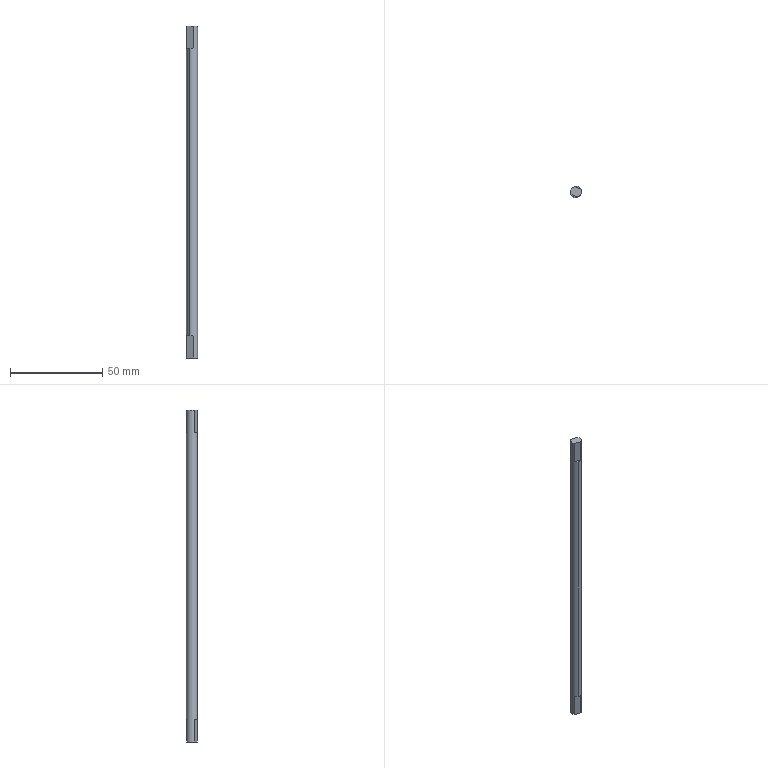Component | SolidWorks | PryBarAxis.1-1 | 1 solid | 12 faces | box 6 x 6 x 180 mm | volume 4991 mm3 | plane 10 | cylinder 2 | commonest cylinder face diameters 6 x2
build123d program:
from build123d import *

# Parameters (mm, degrees)
SKETCH1_R           = 3
BOSS_EXTRUDE1_DEPTH = 180
SKETCH2_W           = 1.83
SKETCH2_H           = 6.945
SKETCH2_W_2         = 2.107
CUT_EXTRUDE1_DEPTH  = 12
SKETCH3_W           = 1.492
SKETCH3_H           = 3.969
SKETCH3_W_2         = 1.313
CUT_EXTRUDE2_DEPTH  = 12


with BuildPart() as part:
    # Sketch1 → Boss-Extrude1 (new body)
    with BuildSketch(Plane.XY):
        with Locations(Location((0, 0, 0), (0, 0, 180))):
            Circle(SKETCH1_R)
    extrude(amount=BOSS_EXTRUDE1_DEPTH)

    # Sketch2 → Cut-Extrude1 (cut)
    with BuildSketch(Plane.XY.offset(180)):
        with Locations((-3.165, 0.1105)):
            Rectangle(SKETCH2_W, SKETCH2_H)
        with Locations((3.303, 0.1105)):
            Rectangle(SKETCH2_W_2, SKETCH2_H)
    extrude(amount=-CUT_EXTRUDE1_DEPTH, mode=Mode.SUBTRACT)

    # Sketch3 → Cut-Extrude2 (cut)
    with BuildSketch(Plane(origin=(0, 0, 0), x_dir=(-1, 0, 0), z_dir=(0, 0, -1))):
        with Locations((2.996, 0)):
            Rectangle(SKETCH3_W, SKETCH3_H)
        with Locations((-2.906, 0)):
            Rectangle(SKETCH3_W_2, SKETCH3_H)
    extrude(amount=-CUT_EXTRUDE2_DEPTH, mode=Mode.SUBTRACT)


solid = part.part

# Placed as in the assembly
solid = solid.moved(Location((65, 200, 90), (-180, 0, -66.765)))
STEP:
#1=COLOUR_RGB('',0.7922,0.8196,0.9333);
#2=FILL_AREA_STYLE_COLOUR('',#1);
#3=FILL_AREA_STYLE('',(#2));
#4=SURFACE_STYLE_FILL_AREA(#3);
#5=SURFACE_SIDE_STYLE('',(#4));
#6=SURFACE_STYLE_USAGE(.BOTH.,#5);
#7=PRESENTATION_STYLE_ASSIGNMENT((#6));
#8=CARTESIAN_POINT('',(2.512,7.765,3.071));
#9=VERTEX_POINT('',#8);
#10=CARTESIAN_POINT('',(2.596,7.762,3.071));
#11=VERTEX_POINT('',#10);
#12=CARTESIAN_POINT('',(2.559,7.874,3.071));
#13=DIRECTION('',(0.,0.,1.));
#14=DIRECTION('',(-0.3945,-0.9189,0.));
#15=AXIS2_PLACEMENT_3D('',#12,#13,#14);
#16=CIRCLE('',#15,0.1181);
#17=EDGE_CURVE('',#9,#11,#16,.T.);
#18=ORIENTED_EDGE('',*,*,#17,.F.);
#19=CARTESIAN_POINT('',(2.512,7.765,-3.071));
#20=VERTEX_POINT('',#19);
#21=CARTESIAN_POINT('',(2.512,7.765,3.543));
#22=DIRECTION('',(0.,0.,-1.));
#23=VECTOR('',#22,39.37);
#24=LINE('',#21,#23);
#25=EDGE_CURVE('',#9,#20,#24,.T.);
#26=ORIENTED_EDGE('',*,*,#25,.T.);
#27=CARTESIAN_POINT('',(2.596,7.762,-3.071));
#28=VERTEX_POINT('',#27);
#29=CARTESIAN_POINT('',(2.559,7.874,-3.071));
#30=DIRECTION('',(0.,0.,-1.));
#31=DIRECTION('',(0.3945,0.9189,0.));
#32=AXIS2_PLACEMENT_3D('',#29,#30,#31);
#33=CIRCLE('',#32,0.1181);
#34=EDGE_CURVE('',#28,#20,#33,.T.);
#35=ORIENTED_EDGE('',*,*,#34,.F.);
#36=CARTESIAN_POINT('',(2.596,7.762,-3.543));
#37=VERTEX_POINT('',#36);
#38=CARTESIAN_POINT('',(2.596,7.762,-3.071));
#39=DIRECTION('',(0.,0.,-1.));
#40=VECTOR('',#39,39.37);
#41=LINE('',#38,#40);
#42=EDGE_CURVE('',#28,#37,#41,.T.);
#43=ORIENTED_EDGE('',*,*,#42,.T.);
#44=CARTESIAN_POINT('',(2.666,7.925,-3.543));
#45=VERTEX_POINT('',#44);
#46=CARTESIAN_POINT('',(2.559,7.874,-3.543));
#47=DIRECTION('',(0.,0.,1.));
#48=DIRECTION('',(-0.3945,-0.9189,0.));
#49=AXIS2_PLACEMENT_3D('',#46,#47,#48);
#50=CIRCLE('',#49,0.1181);
#51=EDGE_CURVE('',#37,#45,#50,.T.);
#52=ORIENTED_EDGE('',*,*,#51,.T.);
#53=CARTESIAN_POINT('',(2.666,7.925,-3.071));
#54=VERTEX_POINT('',#53);
#55=CARTESIAN_POINT('',(2.666,7.925,-3.071));
#56=DIRECTION('',(0.,0.,-1.));
#57=VECTOR('',#56,39.37);
#58=LINE('',#55,#57);
#59=EDGE_CURVE('',#54,#45,#58,.T.);
#60=ORIENTED_EDGE('',*,*,#59,.F.);
#61=CARTESIAN_POINT('',(2.606,7.983,-3.071));
#62=VERTEX_POINT('',#61);
#63=CARTESIAN_POINT('',(2.559,7.874,-3.071));
#64=DIRECTION('',(0.,0.,1.));
#65=DIRECTION('',(-0.3945,-0.9189,0.));
#66=AXIS2_PLACEMENT_3D('',#63,#64,#65);
#67=CIRCLE('',#66,0.1181);
#68=EDGE_CURVE('',#54,#62,#67,.T.);
#69=ORIENTED_EDGE('',*,*,#68,.T.);
#70=CARTESIAN_POINT('',(2.606,7.983,3.071));
#71=VERTEX_POINT('',#70);
#72=CARTESIAN_POINT('',(2.606,7.983,3.543));
#73=DIRECTION('',(0.,0.,-1.));
#74=VECTOR('',#73,39.37);
#75=LINE('',#72,#74);
#76=EDGE_CURVE('',#71,#62,#75,.T.);
#77=ORIENTED_EDGE('',*,*,#76,.F.);
#78=CARTESIAN_POINT('',(2.666,7.925,3.071));
#79=VERTEX_POINT('',#78);
#80=CARTESIAN_POINT('',(2.559,7.874,3.071));
#81=DIRECTION('',(0.,0.,1.));
#82=DIRECTION('',(-0.3945,-0.9189,0.));
#83=AXIS2_PLACEMENT_3D('',#80,#81,#82);
#84=CIRCLE('',#83,0.1181);
#85=EDGE_CURVE('',#79,#71,#84,.T.);
#86=ORIENTED_EDGE('',*,*,#85,.F.);
#87=CARTESIAN_POINT('',(2.666,7.925,3.543));
#88=VERTEX_POINT('',#87);
#89=CARTESIAN_POINT('',(2.666,7.925,3.543));
#90=DIRECTION('',(0.,0.,1.));
#91=VECTOR('',#90,39.37);
#92=LINE('',#89,#91);
#93=EDGE_CURVE('',#79,#88,#92,.T.);
#94=ORIENTED_EDGE('',*,*,#93,.T.);
#95=CARTESIAN_POINT('',(2.596,7.762,3.543));
#96=VERTEX_POINT('',#95);
#97=CARTESIAN_POINT('',(2.559,7.874,3.543));
#98=DIRECTION('',(0.,0.,1.));
#99=DIRECTION('',(-0.3945,-0.9189,0.));
#100=AXIS2_PLACEMENT_3D('',#97,#98,#99);
#101=CIRCLE('',#100,0.1181);
#102=EDGE_CURVE('',#96,#88,#101,.T.);
#103=ORIENTED_EDGE('',*,*,#102,.F.);
#104=CARTESIAN_POINT('',(2.596,7.762,3.543));
#105=DIRECTION('',(0.,0.,-1.));
#106=VECTOR('',#105,39.37);
#107=LINE('',#104,#106);
#108=EDGE_CURVE('',#96,#11,#107,.T.);
#109=ORIENTED_EDGE('',*,*,#108,.T.);
#110=EDGE_LOOP('',(#18,#26,#35,#43,#52,#60,#69,#77,#86,#94,#103,#109));
#111=FACE_OUTER_BOUND('',#110,.T.);
#112=CARTESIAN_POINT('',(2.559,7.874,3.543));
#113=DIRECTION('',(0.,0.,-1.));
#114=DIRECTION('',(0.3945,0.9189,0.));
#115=AXIS2_PLACEMENT_3D('',#112,#113,#114);
#116=CYLINDRICAL_SURFACE('',#115,0.1181);
#117=ADVANCED_FACE('',(#111),#116,.T.);
#118=ORIENTED_EDGE('',*,*,#25,.F.);
#119=CARTESIAN_POINT('',(2.452,7.823,3.071));
#120=VERTEX_POINT('',#119);
#121=CARTESIAN_POINT('',(2.559,7.874,3.071));
#122=DIRECTION('',(0.,0.,1.));
#123=DIRECTION('',(-0.3945,-0.9189,0.));
#124=AXIS2_PLACEMENT_3D('',#121,#122,#123);
#125=CIRCLE('',#124,0.1181);
#126=EDGE_CURVE('',#120,#9,#125,.T.);
#127=ORIENTED_EDGE('',*,*,#126,.F.);
#128=CARTESIAN_POINT('',(2.452,7.823,3.543));
#129=VERTEX_POINT('',#128);
#130=CARTESIAN_POINT('',(2.452,7.823,3.543));
#131=DIRECTION('',(0.,0.,1.));
#132=VECTOR('',#131,39.37);
#133=LINE('',#130,#132);
#134=EDGE_CURVE('',#120,#129,#133,.T.);
#135=ORIENTED_EDGE('',*,*,#134,.T.);
#136=CARTESIAN_POINT('',(2.522,7.986,3.543));
#137=VERTEX_POINT('',#136);
#138=CARTESIAN_POINT('',(2.559,7.874,3.543));
#139=DIRECTION('',(0.,0.,1.));
#140=DIRECTION('',(-0.3945,-0.9189,0.));
#141=AXIS2_PLACEMENT_3D('',#138,#139,#140);
#142=CIRCLE('',#141,0.1181);
#143=EDGE_CURVE('',#137,#129,#142,.T.);
#144=ORIENTED_EDGE('',*,*,#143,.F.);
#145=CARTESIAN_POINT('',(2.522,7.986,3.071));
#146=VERTEX_POINT('',#145);
#147=CARTESIAN_POINT('',(2.522,7.986,3.543));
#148=DIRECTION('',(0.,0.,-1.));
#149=VECTOR('',#148,39.37);
#150=LINE('',#147,#149);
#151=EDGE_CURVE('',#137,#146,#150,.T.);
#152=ORIENTED_EDGE('',*,*,#151,.T.);
#153=CARTESIAN_POINT('',(2.559,7.874,3.071));
#154=DIRECTION('',(0.,0.,1.));
#155=DIRECTION('',(-0.3945,-0.9189,0.));
#156=AXIS2_PLACEMENT_3D('',#153,#154,#155);
#157=CIRCLE('',#156,0.1181);
#158=EDGE_CURVE('',#71,#146,#157,.T.);
#159=ORIENTED_EDGE('',*,*,#158,.F.);
#160=ORIENTED_EDGE('',*,*,#76,.T.);
#161=CARTESIAN_POINT('',(2.522,7.986,-3.071));
#162=VERTEX_POINT('',#161);
#163=CARTESIAN_POINT('',(2.559,7.874,-3.071));
#164=DIRECTION('',(0.,0.,1.));
#165=DIRECTION('',(-0.3945,-0.9189,0.));
#166=AXIS2_PLACEMENT_3D('',#163,#164,#165);
#167=CIRCLE('',#166,0.1181);
#168=EDGE_CURVE('',#62,#162,#167,.T.);
#169=ORIENTED_EDGE('',*,*,#168,.T.);
#170=CARTESIAN_POINT('',(2.522,7.986,-3.543));
#171=VERTEX_POINT('',#170);
#172=CARTESIAN_POINT('',(2.522,7.986,-3.071));
#173=DIRECTION('',(0.,0.,-1.));
#174=VECTOR('',#173,39.37);
#175=LINE('',#172,#174);
#176=EDGE_CURVE('',#162,#171,#175,.T.);
#177=ORIENTED_EDGE('',*,*,#176,.T.);
#178=CARTESIAN_POINT('',(2.452,7.823,-3.543));
#179=VERTEX_POINT('',#178);
#180=CARTESIAN_POINT('',(2.559,7.874,-3.543));
#181=DIRECTION('',(0.,0.,1.));
#182=DIRECTION('',(-0.3945,-0.9189,0.));
#183=AXIS2_PLACEMENT_3D('',#180,#181,#182);
#184=CIRCLE('',#183,0.1181);
#185=EDGE_CURVE('',#171,#179,#184,.T.);
#186=ORIENTED_EDGE('',*,*,#185,.T.);
#187=CARTESIAN_POINT('',(2.452,7.823,-3.071));
#188=VERTEX_POINT('',#187);
#189=CARTESIAN_POINT('',(2.452,7.823,-3.071));
#190=DIRECTION('',(0.,0.,-1.));
#191=VECTOR('',#190,39.37);
#192=LINE('',#189,#191);
#193=EDGE_CURVE('',#188,#179,#192,.T.);
#194=ORIENTED_EDGE('',*,*,#193,.F.);
#195=CARTESIAN_POINT('',(2.559,7.874,-3.071));
#196=DIRECTION('',(0.,0.,-1.));
#197=DIRECTION('',(0.3945,0.9189,0.));
#198=AXIS2_PLACEMENT_3D('',#195,#196,#197);
#199=CIRCLE('',#198,0.1181);
#200=EDGE_CURVE('',#20,#188,#199,.T.);
#201=ORIENTED_EDGE('',*,*,#200,.F.);
#202=EDGE_LOOP('',(#118,#127,#135,#144,#152,#159,#160,#169,#177,#186,#194,#201));
#203=FACE_OUTER_BOUND('',#202,.T.);
#204=CARTESIAN_POINT('',(2.559,7.874,3.543));
#205=DIRECTION('',(0.,0.,-1.));
#206=DIRECTION('',(0.3945,0.9189,0.));
#207=AXIS2_PLACEMENT_3D('',#204,#205,#206);
#208=CYLINDRICAL_SURFACE('',#207,0.1181);
#209=ADVANCED_FACE('',(#203),#208,.T.);
#210=CARTESIAN_POINT('',(2.524,7.793,3.543));
#211=DIRECTION('',(-0.9189,0.3945,0.));
#212=VECTOR('',#211,39.37);
#213=LINE('',#210,#212);
#214=EDGE_CURVE('',#96,#129,#213,.T.);
#215=ORIENTED_EDGE('',*,*,#214,.F.);
#216=ORIENTED_EDGE('',*,*,#102,.T.);
#217=CARTESIAN_POINT('',(2.594,7.955,3.543));
#218=DIRECTION('',(0.9189,-0.3945,0.));
#219=VECTOR('',#218,39.37);
#220=LINE('',#217,#219);
#221=EDGE_CURVE('',#137,#88,#220,.T.);
#222=ORIENTED_EDGE('',*,*,#221,.F.);
#223=ORIENTED_EDGE('',*,*,#143,.T.);
#224=EDGE_LOOP('',(#215,#216,#222,#223));
#225=FACE_OUTER_BOUND('',#224,.T.);
#226=CARTESIAN_POINT('',(2.559,7.874,3.543));
#227=DIRECTION('',(0.,0.,1.));
#228=DIRECTION('',(-0.3945,-0.9189,0.));
#229=AXIS2_PLACEMENT_3D('',#226,#227,#228);
#230=PLANE('',#229);
#231=ADVANCED_FACE('',(#225),#230,.T.);
#232=ORIENTED_EDGE('',*,*,#51,.F.);
#233=CARTESIAN_POINT('',(2.596,7.762,-3.543));
#234=DIRECTION('',(0.9189,-0.3945,0.));
#235=VECTOR('',#234,39.37);
#236=LINE('',#233,#235);
#237=EDGE_CURVE('',#179,#37,#236,.T.);
#238=ORIENTED_EDGE('',*,*,#237,.F.);
#239=ORIENTED_EDGE('',*,*,#185,.F.);
#240=CARTESIAN_POINT('',(2.522,7.986,-3.543));
#241=DIRECTION('',(-0.9189,0.3945,0.));
#242=VECTOR('',#241,39.37);
#243=LINE('',#240,#242);
#244=EDGE_CURVE('',#45,#171,#243,.T.);
#245=ORIENTED_EDGE('',*,*,#244,.F.);
#246=EDGE_LOOP('',(#232,#238,#239,#245));
#247=FACE_OUTER_BOUND('',#246,.T.);
#248=CARTESIAN_POINT('',(2.559,7.874,-3.543));
#249=DIRECTION('',(0.,0.,1.));
#250=DIRECTION('',(-0.3945,-0.9189,0.));
#251=AXIS2_PLACEMENT_3D('',#248,#249,#250);
#252=PLANE('',#251);
#253=ADVANCED_FACE('',(#247),#252,.F.);
#254=ORIENTED_EDGE('',*,*,#85,.T.);
#255=ORIENTED_EDGE('',*,*,#158,.T.);
#256=CARTESIAN_POINT('',(2.724,7.9,3.071));
#257=DIRECTION('',(0.9189,-0.3945,0.));
#258=VECTOR('',#257,39.37);
#259=LINE('',#256,#258);
#260=EDGE_CURVE('',#146,#79,#259,.T.);
#261=ORIENTED_EDGE('',*,*,#260,.T.);
#262=EDGE_LOOP('',(#254,#255,#261));
#263=FACE_OUTER_BOUND('',#262,.T.);
#264=CARTESIAN_POINT('',(2.752,7.966,3.071));
#265=DIRECTION('',(0.,0.,1.));
#266=DIRECTION('',(-0.3945,-0.9189,0.));
#267=AXIS2_PLACEMENT_3D('',#264,#265,#266);
#268=PLANE('',#267);
#269=ADVANCED_FACE('',(#263),#268,.T.);
#270=ORIENTED_EDGE('',*,*,#221,.T.);
#271=ORIENTED_EDGE('',*,*,#93,.F.);
#272=ORIENTED_EDGE('',*,*,#260,.F.);
#273=ORIENTED_EDGE('',*,*,#151,.F.);
#274=EDGE_LOOP('',(#270,#271,#272,#273));
#275=FACE_OUTER_BOUND('',#274,.T.);
#276=CARTESIAN_POINT('',(2.724,7.9,3.071));
#277=DIRECTION('',(-0.3945,-0.9189,0.));
#278=DIRECTION('',(0.9189,-0.3945,0.));
#279=AXIS2_PLACEMENT_3D('',#276,#277,#278);
#280=PLANE('',#279);
#281=ADVANCED_FACE('',(#275),#280,.F.);
#282=ORIENTED_EDGE('',*,*,#126,.T.);
#283=ORIENTED_EDGE('',*,*,#17,.T.);
#284=CARTESIAN_POINT('',(2.654,7.737,3.071));
#285=DIRECTION('',(-0.9189,0.3945,0.));
#286=VECTOR('',#285,39.37);
#287=LINE('',#284,#286);
#288=EDGE_CURVE('',#11,#120,#287,.T.);
#289=ORIENTED_EDGE('',*,*,#288,.T.);
#290=EDGE_LOOP('',(#282,#283,#289));
#291=FACE_OUTER_BOUND('',#290,.T.);
#292=CARTESIAN_POINT('',(2.402,7.845,3.071));
#293=DIRECTION('',(0.,0.,1.));
#294=DIRECTION('',(-0.3945,-0.9189,0.));
#295=AXIS2_PLACEMENT_3D('',#292,#293,#294);
#296=PLANE('',#295);
#297=ADVANCED_FACE('',(#291),#296,.T.);
#298=ORIENTED_EDGE('',*,*,#214,.T.);
#299=ORIENTED_EDGE('',*,*,#134,.F.);
#300=ORIENTED_EDGE('',*,*,#288,.F.);
#301=ORIENTED_EDGE('',*,*,#108,.F.);
#302=EDGE_LOOP('',(#298,#299,#300,#301));
#303=FACE_OUTER_BOUND('',#302,.T.);
#304=CARTESIAN_POINT('',(2.654,7.737,3.071));
#305=DIRECTION('',(0.3945,0.9189,0.));
#306=DIRECTION('',(-0.9189,0.3945,0.));
#307=AXIS2_PLACEMENT_3D('',#304,#305,#306);
#308=PLANE('',#307);
#309=ADVANCED_FACE('',(#303),#308,.F.);
#310=CARTESIAN_POINT('',(2.522,7.986,-3.071));
#311=DIRECTION('',(-0.9189,0.3945,0.));
#312=VECTOR('',#311,39.37);
#313=LINE('',#310,#312);
#314=EDGE_CURVE('',#54,#162,#313,.T.);
#315=ORIENTED_EDGE('',*,*,#314,.T.);
#316=ORIENTED_EDGE('',*,*,#168,.F.);
#317=ORIENTED_EDGE('',*,*,#68,.F.);
#318=EDGE_LOOP('',(#315,#316,#317));
#319=FACE_OUTER_BOUND('',#318,.T.);
#320=CARTESIAN_POINT('',(2.522,7.986,-3.071));
#321=DIRECTION('',(0.,0.,1.));
#322=DIRECTION('',(-0.3945,-0.9189,0.));
#323=AXIS2_PLACEMENT_3D('',#320,#321,#322);
#324=PLANE('',#323);
#325=ADVANCED_FACE('',(#319),#324,.F.);
#326=ORIENTED_EDGE('',*,*,#244,.T.);
#327=ORIENTED_EDGE('',*,*,#176,.F.);
#328=ORIENTED_EDGE('',*,*,#314,.F.);
#329=ORIENTED_EDGE('',*,*,#59,.T.);
#330=EDGE_LOOP('',(#326,#327,#328,#329));
#331=FACE_OUTER_BOUND('',#330,.T.);
#332=CARTESIAN_POINT('',(2.522,7.986,-3.071));
#333=DIRECTION('',(-0.3945,-0.9189,0.));
#334=DIRECTION('',(0.9189,-0.3945,0.));
#335=AXIS2_PLACEMENT_3D('',#332,#333,#334);
#336=PLANE('',#335);
#337=ADVANCED_FACE('',(#331),#336,.F.);
#338=ORIENTED_EDGE('',*,*,#34,.T.);
#339=ORIENTED_EDGE('',*,*,#200,.T.);
#340=CARTESIAN_POINT('',(2.596,7.762,-3.071));
#341=DIRECTION('',(0.9189,-0.3945,0.));
#342=VECTOR('',#341,39.37);
#343=LINE('',#340,#342);
#344=EDGE_CURVE('',#188,#28,#343,.T.);
#345=ORIENTED_EDGE('',*,*,#344,.T.);
#346=EDGE_LOOP('',(#338,#339,#345));
#347=FACE_OUTER_BOUND('',#346,.T.);
#348=CARTESIAN_POINT('',(2.576,7.714,-3.071));
#349=DIRECTION('',(0.,0.,-1.));
#350=DIRECTION('',(0.3945,0.9189,0.));
#351=AXIS2_PLACEMENT_3D('',#348,#349,#350);
#352=PLANE('',#351);
#353=ADVANCED_FACE('',(#347),#352,.T.);
#354=ORIENTED_EDGE('',*,*,#237,.T.);
#355=ORIENTED_EDGE('',*,*,#42,.F.);
#356=ORIENTED_EDGE('',*,*,#344,.F.);
#357=ORIENTED_EDGE('',*,*,#193,.T.);
#358=EDGE_LOOP('',(#354,#355,#356,#357));
#359=FACE_OUTER_BOUND('',#358,.T.);
#360=CARTESIAN_POINT('',(2.596,7.762,-3.071));
#361=DIRECTION('',(0.3945,0.9189,0.));
#362=DIRECTION('',(-0.9189,0.3945,0.));
#363=AXIS2_PLACEMENT_3D('',#360,#361,#362);
#364=PLANE('',#363);
#365=ADVANCED_FACE('',(#359),#364,.F.);
#366=CLOSED_SHELL('',(#117,#209,#231,#253,#269,#281,#297,#309,#325,#337,#353,#365));
#367=MANIFOLD_SOLID_BREP('',#366);
#368=STYLED_ITEM('',(#7),#367);
#369=(LENGTH_UNIT()NAMED_UNIT(*)SI_UNIT($,.METRE.));
#370=LENGTH_MEASURE_WITH_UNIT(LENGTH_MEASURE(0.0254),#369);
#371=DIMENSIONAL_EXPONENTS(1.,0.,0.,0.,0.,0.,0.);
#372=(CONVERSION_BASED_UNIT('',#370)LENGTH_UNIT()NAMED_UNIT(#371));
#373=UNCERTAINTY_MEASURE_WITH_UNIT(LENGTH_MEASURE(0.00001),#372,'','');
#374=(NAMED_UNIT(*)PLANE_ANGLE_UNIT()SI_UNIT($,.RADIAN.));
#375=(NAMED_UNIT(*)SI_UNIT($,.STERADIAN.)SOLID_ANGLE_UNIT());
#376=(GEOMETRIC_REPRESENTATION_CONTEXT(3)GLOBAL_UNCERTAINTY_ASSIGNED_CONTEXT((#373))GLOBAL_UNIT_ASSIGNED_CONTEXT((#372,#374,#375))REPRESENTATION_CONTEXT('',''));
#377=MECHANICAL_DESIGN_GEOMETRIC_PRESENTATION_REPRESENTATION('',(#368),#376);
#378=CARTESIAN_POINT('',(0.,0.,0.));
#379=DIRECTION('',(0.,0.,1.));
#380=DIRECTION('',(1.,0.,0.));
#381=AXIS2_PLACEMENT_3D('',#378,#379,#380);
#382=(LENGTH_UNIT()NAMED_UNIT(*)SI_UNIT($,.METRE.));
#383=LENGTH_MEASURE_WITH_UNIT(LENGTH_MEASURE(0.0254),#382);
#384=DIMENSIONAL_EXPONENTS(1.,0.,0.,0.,0.,0.,0.);
#385=(CONVERSION_BASED_UNIT('',#383)LENGTH_UNIT()NAMED_UNIT(#384));
#386=UNCERTAINTY_MEASURE_WITH_UNIT(LENGTH_MEASURE(0.00001),#385,'','');
#387=(NAMED_UNIT(*)PLANE_ANGLE_UNIT()SI_UNIT($,.RADIAN.));
#388=(NAMED_UNIT(*)SI_UNIT($,.STERADIAN.)SOLID_ANGLE_UNIT());
#389=(GEOMETRIC_REPRESENTATION_CONTEXT(3)GLOBAL_UNCERTAINTY_ASSIGNED_CONTEXT((#386))GLOBAL_UNIT_ASSIGNED_CONTEXT((#385,#387,#388))REPRESENTATION_CONTEXT('',''));
#390=ADVANCED_BREP_SHAPE_REPRESENTATION('',(#367,#381),#389);
#391=PRESENTATION_LAYER_ASSIGNMENT('','',(#368));